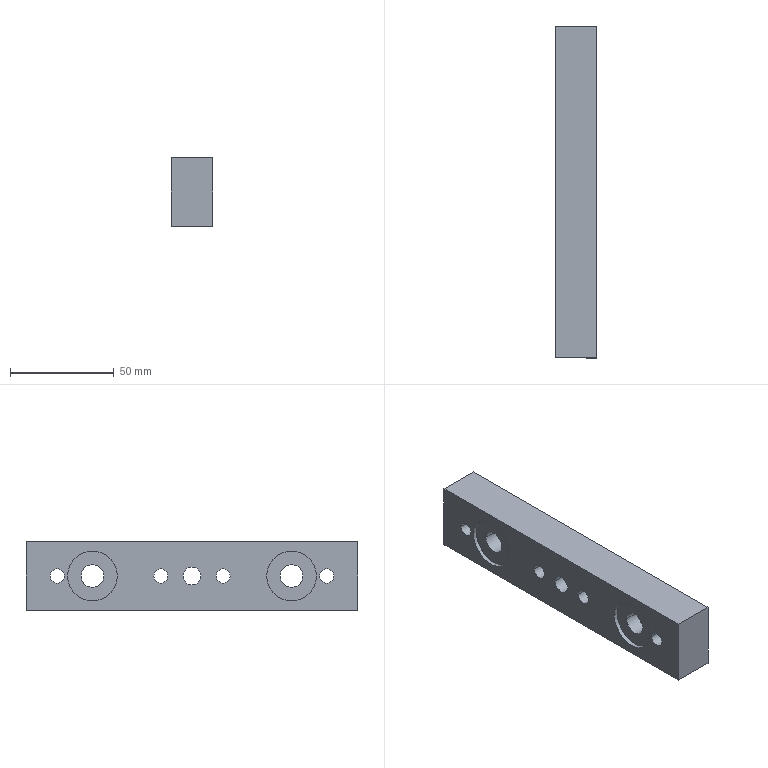Component | SolidWorks | ClampingAssembly-2_CylinderLockingBlock2-1 | 1 solid | 32 faces | box 20 x 160 x 33 mm | volume 92949 mm3 | cylinder 22 | plane 10 | commonest cylinder face diameters 6.8 x8 24 x4 18 x4 11 x4 8.5 x2 | material Q235
build123d program:
from build123d import *

# Parameters (mm, degrees)
SKETCH1_W                                        = 160
SKETCH1_H                                        = 33
BOSS_EXTRUDE1_DEPTH                              = 20
M10_TAPPED_HOLE1_D                               = 8.5
M10_TAPPED_HOLE1_DEPTH                           = 24.5
M10_TAPPED_HOLE1_TIP                             = 2.554
M10_HEX_SOCKET_HEAD_CAP_SCREW_CBORE1_D           = 11
M10_HEX_SOCKET_HEAD_CAP_SCREW_CBORE1_CBORE_D     = 18
M10_HEX_SOCKET_HEAD_CAP_SCREW_CBORE1_CBORE_DEPTH = 10.6
SKETCH7_R                                        = 12
CUT_EXTRUDE1_DEPTH                               = 2
M8_TAPPED_HOLE1_D                                = 6.8


with BuildPart() as part:
    # Sketch1 → Boss-Extrude1 (new body)
    with BuildSketch(Plane.XY):
        Rectangle(SKETCH1_W, SKETCH1_H)
    extrude(amount=BOSS_EXTRUDE1_DEPTH)

    # M10 Tapped Hole1
    with Locations(Plane.XY.offset(20)):
        with Locations((0, 0)):
            Hole(M10_TAPPED_HOLE1_D / 2, depth=M10_TAPPED_HOLE1_DEPTH)
            with Locations((0, 0, -(M10_TAPPED_HOLE1_DEPTH + M10_TAPPED_HOLE1_TIP / 2))):  # 118° drill point
                Cone(0, M10_TAPPED_HOLE1_D / 2, M10_TAPPED_HOLE1_TIP, mode=Mode.SUBTRACT)

    # M10 Hex Socket Head Cap Screw CBORE1 (through all)
    with Locations(Plane(origin=(-48, 0, 0), x_dir=(-1, 0, 0), z_dir=(0, 0, -1))):
        with Locations((0, 0)):
            m10_hex_socket_head_cap_screw_cbore1 = CounterBoreHole(M10_HEX_SOCKET_HEAD_CAP_SCREW_CBORE1_D / 2, M10_HEX_SOCKET_HEAD_CAP_SCREW_CBORE1_CBORE_D / 2, M10_HEX_SOCKET_HEAD_CAP_SCREW_CBORE1_CBORE_DEPTH)

    # Mirror1: M10 Hex Socket Head Cap Screw CBORE1 across plane
    add(m10_hex_socket_head_cap_screw_cbore1.mirror(Plane(origin=(0, 0, 0), x_dir=(0, 0, 1), z_dir=(1, 0, 0))), mode=Mode.SUBTRACT)

    # Sketch7 → Cut-Extrude1 (cut)
    with BuildSketch(Plane.XY.offset(20)):
        with Locations((-48, 0)):
            Circle(SKETCH7_R)
        with Locations((48, 0)):
            Circle(SKETCH7_R)
    extrude(amount=-CUT_EXTRUDE1_DEPTH, mode=Mode.SUBTRACT)

    # M8 Tapped Hole1 (through all)
    with Locations(Plane(origin=(65, 0, 0), x_dir=(-1, 0, 0), z_dir=(0, 0, -1))):
        with Locations((0, 0), (50, 0), (80, 0), (130, 0)):
            Hole(M8_TAPPED_HOLE1_D / 2)


solid = part.part

# Placed as in the assembly
solid = solid.moved(Location((-116.365, -26.917, -1210.457), (90, -90, 0)))
STEP:
#1=COLOUR_RGB('',0.7922,0.8196,0.9333);
#2=FILL_AREA_STYLE_COLOUR('',#1);
#3=FILL_AREA_STYLE('',(#2));
#4=SURFACE_STYLE_FILL_AREA(#3);
#5=SURFACE_SIDE_STYLE('',(#4));
#6=SURFACE_STYLE_USAGE(.BOTH.,#5);
#7=PRESENTATION_STYLE_ASSIGNMENT((#6));
#8=CARTESIAN_POINT('',(-5.369,-3.753,-47.656));
#9=VERTEX_POINT('',#8);
#10=CARTESIAN_POINT('',(-5.369,-3.485,-47.656));
#11=VERTEX_POINT('',#10);
#12=CARTESIAN_POINT('',(-5.369,-3.619,-47.656));
#13=DIRECTION('',(1.,-0.,0.));
#14=DIRECTION('',(0.,1.,0.));
#15=AXIS2_PLACEMENT_3D('',#12,#13,#14);
#16=CIRCLE('',#15,0.1339);
#17=EDGE_CURVE('',#9,#11,#16,.T.);
#18=ORIENTED_EDGE('',*,*,#17,.F.);
#19=CARTESIAN_POINT('',(-4.581,-3.753,-47.656));
#20=VERTEX_POINT('',#19);
#21=CARTESIAN_POINT('',(-4.581,-3.753,-47.656));
#22=DIRECTION('',(1.,-0.,0.));
#23=VECTOR('',#22,39.37);
#24=LINE('',#21,#23);
#25=EDGE_CURVE('',#9,#20,#24,.T.);
#26=ORIENTED_EDGE('',*,*,#25,.T.);
#27=CARTESIAN_POINT('',(-4.581,-3.485,-47.656));
#28=VERTEX_POINT('',#27);
#29=CARTESIAN_POINT('',(-4.581,-3.619,-47.656));
#30=DIRECTION('',(1.,-0.,0.));
#31=DIRECTION('',(0.,1.,0.));
#32=AXIS2_PLACEMENT_3D('',#29,#30,#31);
#33=CIRCLE('',#32,0.1339);
#34=EDGE_CURVE('',#20,#28,#33,.T.);
#35=ORIENTED_EDGE('',*,*,#34,.T.);
#36=CARTESIAN_POINT('',(-4.581,-3.485,-47.656));
#37=DIRECTION('',(1.,-0.,0.));
#38=VECTOR('',#37,39.37);
#39=LINE('',#36,#38);
#40=EDGE_CURVE('',#11,#28,#39,.T.);
#41=ORIENTED_EDGE('',*,*,#40,.F.);
#42=EDGE_LOOP('',(#18,#26,#35,#41));
#43=FACE_OUTER_BOUND('',#42,.T.);
#44=CARTESIAN_POINT('',(-4.581,-3.619,-47.656));
#45=DIRECTION('',(1.,-0.,0.));
#46=DIRECTION('',(0.,1.,0.));
#47=AXIS2_PLACEMENT_3D('',#44,#45,#46);
#48=CYLINDRICAL_SURFACE('',#47,0.1339);
#49=ADVANCED_FACE('',(#43),#48,.F.);
#50=CARTESIAN_POINT('',(-5.369,-1.784,-47.656));
#51=VERTEX_POINT('',#50);
#52=CARTESIAN_POINT('',(-5.369,-1.516,-47.656));
#53=VERTEX_POINT('',#52);
#54=CARTESIAN_POINT('',(-5.369,-1.65,-47.656));
#55=DIRECTION('',(1.,-0.,0.));
#56=DIRECTION('',(0.,1.,0.));
#57=AXIS2_PLACEMENT_3D('',#54,#55,#56);
#58=CIRCLE('',#57,0.1339);
#59=EDGE_CURVE('',#51,#53,#58,.T.);
#60=ORIENTED_EDGE('',*,*,#59,.F.);
#61=CARTESIAN_POINT('',(-4.581,-1.784,-47.656));
#62=VERTEX_POINT('',#61);
#63=CARTESIAN_POINT('',(-4.581,-1.784,-47.656));
#64=DIRECTION('',(1.,-0.,0.));
#65=VECTOR('',#64,39.37);
#66=LINE('',#63,#65);
#67=EDGE_CURVE('',#51,#62,#66,.T.);
#68=ORIENTED_EDGE('',*,*,#67,.T.);
#69=CARTESIAN_POINT('',(-4.581,-1.516,-47.656));
#70=VERTEX_POINT('',#69);
#71=CARTESIAN_POINT('',(-4.581,-1.65,-47.656));
#72=DIRECTION('',(1.,-0.,0.));
#73=DIRECTION('',(0.,1.,0.));
#74=AXIS2_PLACEMENT_3D('',#71,#72,#73);
#75=CIRCLE('',#74,0.1339);
#76=EDGE_CURVE('',#62,#70,#75,.T.);
#77=ORIENTED_EDGE('',*,*,#76,.T.);
#78=CARTESIAN_POINT('',(-4.581,-1.516,-47.656));
#79=DIRECTION('',(1.,-0.,0.));
#80=VECTOR('',#79,39.37);
#81=LINE('',#78,#80);
#82=EDGE_CURVE('',#53,#70,#81,.T.);
#83=ORIENTED_EDGE('',*,*,#82,.F.);
#84=EDGE_LOOP('',(#60,#68,#77,#83));
#85=FACE_OUTER_BOUND('',#84,.T.);
#86=CARTESIAN_POINT('',(-4.581,-1.65,-47.656));
#87=DIRECTION('',(1.,-0.,0.));
#88=DIRECTION('',(0.,1.,0.));
#89=AXIS2_PLACEMENT_3D('',#86,#87,#88);
#90=CYLINDRICAL_SURFACE('',#89,0.1339);
#91=ADVANCED_FACE('',(#85),#90,.F.);
#92=CARTESIAN_POINT('',(-5.369,-0.603,-47.656));
#93=VERTEX_POINT('',#92);
#94=CARTESIAN_POINT('',(-5.369,-0.3353,-47.656));
#95=VERTEX_POINT('',#94);
#96=CARTESIAN_POINT('',(-5.369,-0.4692,-47.656));
#97=DIRECTION('',(1.,-0.,0.));
#98=DIRECTION('',(0.,1.,0.));
#99=AXIS2_PLACEMENT_3D('',#96,#97,#98);
#100=CIRCLE('',#99,0.1339);
#101=EDGE_CURVE('',#93,#95,#100,.T.);
#102=ORIENTED_EDGE('',*,*,#101,.F.);
#103=CARTESIAN_POINT('',(-4.581,-0.603,-47.656));
#104=VERTEX_POINT('',#103);
#105=CARTESIAN_POINT('',(-4.581,-0.603,-47.656));
#106=DIRECTION('',(1.,-0.,0.));
#107=VECTOR('',#106,39.37);
#108=LINE('',#105,#107);
#109=EDGE_CURVE('',#93,#104,#108,.T.);
#110=ORIENTED_EDGE('',*,*,#109,.T.);
#111=CARTESIAN_POINT('',(-4.581,-0.3353,-47.656));
#112=VERTEX_POINT('',#111);
#113=CARTESIAN_POINT('',(-4.581,-0.4692,-47.656));
#114=DIRECTION('',(1.,-0.,0.));
#115=DIRECTION('',(0.,1.,0.));
#116=AXIS2_PLACEMENT_3D('',#113,#114,#115);
#117=CIRCLE('',#116,0.1339);
#118=EDGE_CURVE('',#104,#112,#117,.T.);
#119=ORIENTED_EDGE('',*,*,#118,.T.);
#120=CARTESIAN_POINT('',(-4.581,-0.3353,-47.656));
#121=DIRECTION('',(1.,-0.,0.));
#122=VECTOR('',#121,39.37);
#123=LINE('',#120,#122);
#124=EDGE_CURVE('',#95,#112,#123,.T.);
#125=ORIENTED_EDGE('',*,*,#124,.F.);
#126=EDGE_LOOP('',(#102,#110,#119,#125));
#127=FACE_OUTER_BOUND('',#126,.T.);
#128=CARTESIAN_POINT('',(-4.581,-0.4692,-47.656));
#129=DIRECTION('',(1.,-0.,0.));
#130=DIRECTION('',(0.,1.,0.));
#131=AXIS2_PLACEMENT_3D('',#128,#129,#130);
#132=CYLINDRICAL_SURFACE('',#131,0.1339);
#133=ADVANCED_FACE('',(#127),#132,.F.);
#134=CARTESIAN_POINT('',(-5.369,1.365,-47.656));
#135=VERTEX_POINT('',#134);
#136=CARTESIAN_POINT('',(-5.369,1.633,-47.656));
#137=VERTEX_POINT('',#136);
#138=CARTESIAN_POINT('',(-5.369,1.499,-47.656));
#139=DIRECTION('',(1.,-0.,0.));
#140=DIRECTION('',(0.,1.,0.));
#141=AXIS2_PLACEMENT_3D('',#138,#139,#140);
#142=CIRCLE('',#141,0.1339);
#143=EDGE_CURVE('',#135,#137,#142,.T.);
#144=ORIENTED_EDGE('',*,*,#143,.F.);
#145=CARTESIAN_POINT('',(-4.581,1.365,-47.656));
#146=VERTEX_POINT('',#145);
#147=CARTESIAN_POINT('',(-4.581,1.365,-47.656));
#148=DIRECTION('',(1.,-0.,0.));
#149=VECTOR('',#148,39.37);
#150=LINE('',#147,#149);
#151=EDGE_CURVE('',#135,#146,#150,.T.);
#152=ORIENTED_EDGE('',*,*,#151,.T.);
#153=CARTESIAN_POINT('',(-4.581,1.633,-47.656));
#154=VERTEX_POINT('',#153);
#155=CARTESIAN_POINT('',(-4.581,1.499,-47.656));
#156=DIRECTION('',(1.,-0.,0.));
#157=DIRECTION('',(0.,1.,0.));
#158=AXIS2_PLACEMENT_3D('',#155,#156,#157);
#159=CIRCLE('',#158,0.1339);
#160=EDGE_CURVE('',#146,#154,#159,.T.);
#161=ORIENTED_EDGE('',*,*,#160,.T.);
#162=CARTESIAN_POINT('',(-4.581,1.633,-47.656));
#163=DIRECTION('',(1.,-0.,0.));
#164=VECTOR('',#163,39.37);
#165=LINE('',#162,#164);
#166=EDGE_CURVE('',#137,#154,#165,.T.);
#167=ORIENTED_EDGE('',*,*,#166,.F.);
#168=EDGE_LOOP('',(#144,#152,#161,#167));
#169=FACE_OUTER_BOUND('',#168,.T.);
#170=CARTESIAN_POINT('',(-4.581,1.499,-47.656));
#171=DIRECTION('',(1.,-0.,0.));
#172=DIRECTION('',(0.,1.,0.));
#173=AXIS2_PLACEMENT_3D('',#170,#171,#172);
#174=CYLINDRICAL_SURFACE('',#173,0.1339);
#175=ADVANCED_FACE('',(#169),#174,.F.);
#176=CARTESIAN_POINT('',(-5.29,-2.477,-47.656));
#177=VERTEX_POINT('',#176);
#178=CARTESIAN_POINT('',(-5.29,-3.422,-47.656));
#179=VERTEX_POINT('',#178);
#180=CARTESIAN_POINT('',(-5.29,-2.949,-47.656));
#181=DIRECTION('',(-1.,0.,-0.));
#182=DIRECTION('',(0.,-1.,0.));
#183=AXIS2_PLACEMENT_3D('',#180,#181,#182);
#184=CIRCLE('',#183,0.4724);
#185=EDGE_CURVE('',#177,#179,#184,.T.);
#186=ORIENTED_EDGE('',*,*,#185,.F.);
#187=CARTESIAN_POINT('',(-5.369,-2.477,-47.656));
#188=VERTEX_POINT('',#187);
#189=CARTESIAN_POINT('',(-5.29,-2.477,-47.656));
#190=DIRECTION('',(-1.,0.,-0.));
#191=VECTOR('',#190,39.37);
#192=LINE('',#189,#191);
#193=EDGE_CURVE('',#177,#188,#192,.T.);
#194=ORIENTED_EDGE('',*,*,#193,.T.);
#195=CARTESIAN_POINT('',(-5.369,-3.422,-47.656));
#196=VERTEX_POINT('',#195);
#197=CARTESIAN_POINT('',(-5.369,-2.949,-47.656));
#198=DIRECTION('',(-1.,0.,-0.));
#199=DIRECTION('',(0.,-1.,0.));
#200=AXIS2_PLACEMENT_3D('',#197,#198,#199);
#201=CIRCLE('',#200,0.4724);
#202=EDGE_CURVE('',#188,#196,#201,.T.);
#203=ORIENTED_EDGE('',*,*,#202,.T.);
#204=CARTESIAN_POINT('',(-5.29,-3.422,-47.656));
#205=DIRECTION('',(-1.,0.,-0.));
#206=VECTOR('',#205,39.37);
#207=LINE('',#204,#206);
#208=EDGE_CURVE('',#179,#196,#207,.T.);
#209=ORIENTED_EDGE('',*,*,#208,.F.);
#210=EDGE_LOOP('',(#186,#194,#203,#209));
#211=FACE_OUTER_BOUND('',#210,.T.);
#212=CARTESIAN_POINT('',(-5.29,-2.949,-47.656));
#213=DIRECTION('',(-1.,0.,-0.));
#214=DIRECTION('',(0.,-1.,0.));
#215=AXIS2_PLACEMENT_3D('',#212,#213,#214);
#216=CYLINDRICAL_SURFACE('',#215,0.4724);
#217=ADVANCED_FACE('',(#211),#216,.F.);
#218=CARTESIAN_POINT('',(-5.29,1.302,-47.656));
#219=VERTEX_POINT('',#218);
#220=CARTESIAN_POINT('',(-5.29,0.3576,-47.656));
#221=VERTEX_POINT('',#220);
#222=CARTESIAN_POINT('',(-5.29,0.83,-47.656));
#223=DIRECTION('',(-1.,0.,-0.));
#224=DIRECTION('',(0.,-1.,0.));
#225=AXIS2_PLACEMENT_3D('',#222,#223,#224);
#226=CIRCLE('',#225,0.4724);
#227=EDGE_CURVE('',#219,#221,#226,.T.);
#228=ORIENTED_EDGE('',*,*,#227,.F.);
#229=CARTESIAN_POINT('',(-5.369,1.302,-47.656));
#230=VERTEX_POINT('',#229);
#231=CARTESIAN_POINT('',(-5.29,1.302,-47.656));
#232=DIRECTION('',(-1.,0.,-0.));
#233=VECTOR('',#232,39.37);
#234=LINE('',#231,#233);
#235=EDGE_CURVE('',#219,#230,#234,.T.);
#236=ORIENTED_EDGE('',*,*,#235,.T.);
#237=CARTESIAN_POINT('',(-5.369,0.3576,-47.656));
#238=VERTEX_POINT('',#237);
#239=CARTESIAN_POINT('',(-5.369,0.83,-47.656));
#240=DIRECTION('',(-1.,0.,-0.));
#241=DIRECTION('',(0.,-1.,0.));
#242=AXIS2_PLACEMENT_3D('',#239,#240,#241);
#243=CIRCLE('',#242,0.4724);
#244=EDGE_CURVE('',#230,#238,#243,.T.);
#245=ORIENTED_EDGE('',*,*,#244,.T.);
#246=CARTESIAN_POINT('',(-5.29,0.3576,-47.656));
#247=DIRECTION('',(-1.,0.,-0.));
#248=VECTOR('',#247,39.37);
#249=LINE('',#246,#248);
#250=EDGE_CURVE('',#221,#238,#249,.T.);
#251=ORIENTED_EDGE('',*,*,#250,.F.);
#252=EDGE_LOOP('',(#228,#236,#245,#251));
#253=FACE_OUTER_BOUND('',#252,.T.);
#254=CARTESIAN_POINT('',(-5.29,0.83,-47.656));
#255=DIRECTION('',(-1.,0.,-0.));
#256=DIRECTION('',(0.,-1.,0.));
#257=AXIS2_PLACEMENT_3D('',#254,#255,#256);
#258=CYLINDRICAL_SURFACE('',#257,0.4724);
#259=ADVANCED_FACE('',(#253),#258,.F.);
#260=CARTESIAN_POINT('',(-4.999,-3.304,-47.656));
#261=VERTEX_POINT('',#260);
#262=CARTESIAN_POINT('',(-4.999,-2.595,-47.656));
#263=VERTEX_POINT('',#262);
#264=CARTESIAN_POINT('',(-4.999,-2.949,-47.656));
#265=DIRECTION('',(1.,-0.,0.));
#266=DIRECTION('',(0.,1.,0.));
#267=AXIS2_PLACEMENT_3D('',#264,#265,#266);
#268=CIRCLE('',#267,0.3543);
#269=EDGE_CURVE('',#261,#263,#268,.T.);
#270=ORIENTED_EDGE('',*,*,#269,.F.);
#271=CARTESIAN_POINT('',(-4.581,-3.304,-47.656));
#272=VERTEX_POINT('',#271);
#273=CARTESIAN_POINT('',(-4.581,-3.304,-47.656));
#274=DIRECTION('',(1.,-0.,0.));
#275=VECTOR('',#274,39.37);
#276=LINE('',#273,#275);
#277=EDGE_CURVE('',#261,#272,#276,.T.);
#278=ORIENTED_EDGE('',*,*,#277,.T.);
#279=CARTESIAN_POINT('',(-4.581,-2.595,-47.656));
#280=VERTEX_POINT('',#279);
#281=CARTESIAN_POINT('',(-4.581,-2.949,-47.656));
#282=DIRECTION('',(1.,-0.,0.));
#283=DIRECTION('',(0.,1.,0.));
#284=AXIS2_PLACEMENT_3D('',#281,#282,#283);
#285=CIRCLE('',#284,0.3543);
#286=EDGE_CURVE('',#272,#280,#285,.T.);
#287=ORIENTED_EDGE('',*,*,#286,.T.);
#288=CARTESIAN_POINT('',(-4.581,-2.595,-47.656));
#289=DIRECTION('',(1.,-0.,0.));
#290=VECTOR('',#289,39.37);
#291=LINE('',#288,#290);
#292=EDGE_CURVE('',#263,#280,#291,.T.);
#293=ORIENTED_EDGE('',*,*,#292,.F.);
#294=EDGE_LOOP('',(#270,#278,#287,#293));
#295=FACE_OUTER_BOUND('',#294,.T.);
#296=CARTESIAN_POINT('',(-4.581,-2.949,-47.656));
#297=DIRECTION('',(1.,-0.,0.));
#298=DIRECTION('',(0.,1.,0.));
#299=AXIS2_PLACEMENT_3D('',#296,#297,#298);
#300=CYLINDRICAL_SURFACE('',#299,0.3543);
#301=ADVANCED_FACE('',(#295),#300,.F.);
#302=CARTESIAN_POINT('',(-4.999,0.4757,-47.656));
#303=VERTEX_POINT('',#302);
#304=CARTESIAN_POINT('',(-4.999,1.184,-47.656));
#305=VERTEX_POINT('',#304);
#306=CARTESIAN_POINT('',(-4.999,0.83,-47.656));
#307=DIRECTION('',(1.,-0.,0.));
#308=DIRECTION('',(0.,1.,0.));
#309=AXIS2_PLACEMENT_3D('',#306,#307,#308);
#310=CIRCLE('',#309,0.3543);
#311=EDGE_CURVE('',#303,#305,#310,.T.);
#312=ORIENTED_EDGE('',*,*,#311,.F.);
#313=CARTESIAN_POINT('',(-4.581,0.4757,-47.656));
#314=VERTEX_POINT('',#313);
#315=CARTESIAN_POINT('',(-4.581,0.4757,-47.656));
#316=DIRECTION('',(1.,-0.,0.));
#317=VECTOR('',#316,39.37);
#318=LINE('',#315,#317);
#319=EDGE_CURVE('',#303,#314,#318,.T.);
#320=ORIENTED_EDGE('',*,*,#319,.T.);
#321=CARTESIAN_POINT('',(-4.581,1.184,-47.656));
#322=VERTEX_POINT('',#321);
#323=CARTESIAN_POINT('',(-4.581,0.83,-47.656));
#324=DIRECTION('',(1.,-0.,0.));
#325=DIRECTION('',(0.,1.,0.));
#326=AXIS2_PLACEMENT_3D('',#323,#324,#325);
#327=CIRCLE('',#326,0.3543);
#328=EDGE_CURVE('',#314,#322,#327,.T.);
#329=ORIENTED_EDGE('',*,*,#328,.T.);
#330=CARTESIAN_POINT('',(-4.581,1.184,-47.656));
#331=DIRECTION('',(1.,-0.,0.));
#332=VECTOR('',#331,39.37);
#333=LINE('',#330,#332);
#334=EDGE_CURVE('',#305,#322,#333,.T.);
#335=ORIENTED_EDGE('',*,*,#334,.F.);
#336=EDGE_LOOP('',(#312,#320,#329,#335));
#337=FACE_OUTER_BOUND('',#336,.T.);
#338=CARTESIAN_POINT('',(-4.581,0.83,-47.656));
#339=DIRECTION('',(1.,-0.,0.));
#340=DIRECTION('',(0.,1.,0.));
#341=AXIS2_PLACEMENT_3D('',#338,#339,#340);
#342=CYLINDRICAL_SURFACE('',#341,0.3543);
#343=ADVANCED_FACE('',(#337),#342,.F.);
#344=CARTESIAN_POINT('',(-4.581,-0.8924,-47.656));
#345=VERTEX_POINT('',#344);
#346=CARTESIAN_POINT('',(-4.581,-1.227,-47.656));
#347=VERTEX_POINT('',#346);
#348=CARTESIAN_POINT('',(-4.581,-1.06,-47.656));
#349=DIRECTION('',(-1.,0.,-0.));
#350=DIRECTION('',(0.,-1.,0.));
#351=AXIS2_PLACEMENT_3D('',#348,#349,#350);
#352=CIRCLE('',#351,0.1673);
#353=EDGE_CURVE('',#345,#347,#352,.T.);
#354=ORIENTED_EDGE('',*,*,#353,.F.);
#355=CARTESIAN_POINT('',(-5.369,-0.8924,-47.656));
#356=VERTEX_POINT('',#355);
#357=CARTESIAN_POINT('',(-5.369,-0.8924,-47.656));
#358=DIRECTION('',(-1.,0.,-0.));
#359=VECTOR('',#358,39.37);
#360=LINE('',#357,#359);
#361=EDGE_CURVE('',#345,#356,#360,.T.);
#362=ORIENTED_EDGE('',*,*,#361,.T.);
#363=CARTESIAN_POINT('',(-5.369,-1.227,-47.656));
#364=VERTEX_POINT('',#363);
#365=CARTESIAN_POINT('',(-5.369,-1.06,-47.656));
#366=DIRECTION('',(-1.,0.,-0.));
#367=DIRECTION('',(0.,-1.,0.));
#368=AXIS2_PLACEMENT_3D('',#365,#366,#367);
#369=CIRCLE('',#368,0.1673);
#370=EDGE_CURVE('',#356,#364,#369,.T.);
#371=ORIENTED_EDGE('',*,*,#370,.T.);
#372=CARTESIAN_POINT('',(-5.369,-1.227,-47.656));
#373=DIRECTION('',(-1.,0.,-0.));
#374=VECTOR('',#373,39.37);
#375=LINE('',#372,#374);
#376=EDGE_CURVE('',#347,#364,#375,.T.);
#377=ORIENTED_EDGE('',*,*,#376,.F.);
#378=EDGE_LOOP('',(#354,#362,#371,#377));
#379=FACE_OUTER_BOUND('',#378,.T.);
#380=CARTESIAN_POINT('',(-5.369,-1.06,-47.656));
#381=DIRECTION('',(-1.,0.,-0.));
#382=DIRECTION('',(0.,-1.,0.));
#383=AXIS2_PLACEMENT_3D('',#380,#381,#382);
#384=CYLINDRICAL_SURFACE('',#383,0.1673);
#385=ADVANCED_FACE('',(#379),#384,.F.);
#386=CARTESIAN_POINT('',(-5.29,0.6135,-47.656));
#387=VERTEX_POINT('',#386);
#388=CARTESIAN_POINT('',(-5.29,1.047,-47.656));
#389=VERTEX_POINT('',#388);
#390=CARTESIAN_POINT('',(-5.29,0.83,-47.656));
#391=DIRECTION('',(1.,-0.,0.));
#392=DIRECTION('',(0.,-1.,0.));
#393=AXIS2_PLACEMENT_3D('',#390,#391,#392);
#394=CIRCLE('',#393,0.2165);
#395=EDGE_CURVE('',#387,#389,#394,.T.);
#396=ORIENTED_EDGE('',*,*,#395,.F.);
#397=CARTESIAN_POINT('',(-4.999,0.6135,-47.656));
#398=VERTEX_POINT('',#397);
#399=CARTESIAN_POINT('',(-4.581,0.6135,-47.656));
#400=DIRECTION('',(1.,-0.,0.));
#401=VECTOR('',#400,39.37);
#402=LINE('',#399,#401);
#403=EDGE_CURVE('',#387,#398,#402,.T.);
#404=ORIENTED_EDGE('',*,*,#403,.T.);
#405=CARTESIAN_POINT('',(-4.999,1.047,-47.656));
#406=VERTEX_POINT('',#405);
#407=CARTESIAN_POINT('',(-4.999,0.83,-47.656));
#408=DIRECTION('',(1.,-0.,0.));
#409=DIRECTION('',(0.,1.,0.));
#410=AXIS2_PLACEMENT_3D('',#407,#408,#409);
#411=CIRCLE('',#410,0.2165);
#412=EDGE_CURVE('',#398,#406,#411,.T.);
#413=ORIENTED_EDGE('',*,*,#412,.T.);
#414=CARTESIAN_POINT('',(-4.581,1.047,-47.656));
#415=DIRECTION('',(1.,-0.,0.));
#416=VECTOR('',#415,39.37);
#417=LINE('',#414,#416);
#418=EDGE_CURVE('',#389,#406,#417,.T.);
#419=ORIENTED_EDGE('',*,*,#418,.F.);
#420=EDGE_LOOP('',(#396,#404,#413,#419));
#421=FACE_OUTER_BOUND('',#420,.T.);
#422=CARTESIAN_POINT('',(-4.581,0.83,-47.656));
#423=DIRECTION('',(1.,-0.,0.));
#424=DIRECTION('',(0.,1.,0.));
#425=AXIS2_PLACEMENT_3D('',#422,#423,#424);
#426=CYLINDRICAL_SURFACE('',#425,0.2165);
#427=ADVANCED_FACE('',(#421),#426,.F.);
#428=CARTESIAN_POINT('',(-5.29,-3.166,-47.656));
#429=VERTEX_POINT('',#428);
#430=CARTESIAN_POINT('',(-5.29,-2.733,-47.656));
#431=VERTEX_POINT('',#430);
#432=CARTESIAN_POINT('',(-5.29,-2.949,-47.656));
#433=DIRECTION('',(1.,-0.,0.));
#434=DIRECTION('',(0.,-1.,0.));
#435=AXIS2_PLACEMENT_3D('',#432,#433,#434);
#436=CIRCLE('',#435,0.2165);
#437=EDGE_CURVE('',#429,#431,#436,.T.);
#438=ORIENTED_EDGE('',*,*,#437,.F.);
#439=CARTESIAN_POINT('',(-4.999,-3.166,-47.656));
#440=VERTEX_POINT('',#439);
#441=CARTESIAN_POINT('',(-4.581,-3.166,-47.656));
#442=DIRECTION('',(1.,-0.,0.));
#443=VECTOR('',#442,39.37);
#444=LINE('',#441,#443);
#445=EDGE_CURVE('',#429,#440,#444,.T.);
#446=ORIENTED_EDGE('',*,*,#445,.T.);
#447=CARTESIAN_POINT('',(-4.999,-2.733,-47.656));
#448=VERTEX_POINT('',#447);
#449=CARTESIAN_POINT('',(-4.999,-2.949,-47.656));
#450=DIRECTION('',(1.,-0.,0.));
#451=DIRECTION('',(0.,1.,0.));
#452=AXIS2_PLACEMENT_3D('',#449,#450,#451);
#453=CIRCLE('',#452,0.2165);
#454=EDGE_CURVE('',#440,#448,#453,.T.);
#455=ORIENTED_EDGE('',*,*,#454,.T.);
#456=CARTESIAN_POINT('',(-4.581,-2.733,-47.656));
#457=DIRECTION('',(1.,-0.,0.));
#458=VECTOR('',#457,39.37);
#459=LINE('',#456,#458);
#460=EDGE_CURVE('',#431,#448,#459,.T.);
#461=ORIENTED_EDGE('',*,*,#460,.F.);
#462=EDGE_LOOP('',(#438,#446,#455,#461));
#463=FACE_OUTER_BOUND('',#462,.T.);
#464=CARTESIAN_POINT('',(-4.581,-2.949,-47.656));
#465=DIRECTION('',(1.,-0.,0.));
#466=DIRECTION('',(0.,1.,0.));
#467=AXIS2_PLACEMENT_3D('',#464,#465,#466);
#468=CYLINDRICAL_SURFACE('',#467,0.2165);
#469=ADVANCED_FACE('',(#463),#468,.F.);
#470=ORIENTED_EDGE('',*,*,#445,.F.);
#471=CARTESIAN_POINT('',(-5.29,-2.949,-47.656));
#472=DIRECTION('',(1.,-0.,0.));
#473=DIRECTION('',(0.,-1.,0.));
#474=AXIS2_PLACEMENT_3D('',#471,#472,#473);
#475=CIRCLE('',#474,0.2165);
#476=EDGE_CURVE('',#431,#429,#475,.T.);
#477=ORIENTED_EDGE('',*,*,#476,.F.);
#478=ORIENTED_EDGE('',*,*,#460,.T.);
#479=CARTESIAN_POINT('',(-4.999,-2.949,-47.656));
#480=DIRECTION('',(1.,-0.,0.));
#481=DIRECTION('',(0.,1.,0.));
#482=AXIS2_PLACEMENT_3D('',#479,#480,#481);
#483=CIRCLE('',#482,0.2165);
#484=EDGE_CURVE('',#448,#440,#483,.T.);
#485=ORIENTED_EDGE('',*,*,#484,.T.);
#486=EDGE_LOOP('',(#470,#477,#478,#485));
#487=FACE_OUTER_BOUND('',#486,.T.);
#488=CARTESIAN_POINT('',(-4.581,-2.949,-47.656));
#489=DIRECTION('',(1.,-0.,0.));
#490=DIRECTION('',(0.,1.,0.));
#491=AXIS2_PLACEMENT_3D('',#488,#489,#490);
#492=CYLINDRICAL_SURFACE('',#491,0.2165);
#493=ADVANCED_FACE('',(#487),#492,.F.);
#494=ORIENTED_EDGE('',*,*,#403,.F.);
#495=CARTESIAN_POINT('',(-5.29,0.83,-47.656));
#496=DIRECTION('',(1.,-0.,0.));
#497=DIRECTION('',(0.,-1.,0.));
#498=AXIS2_PLACEMENT_3D('',#495,#496,#497);
#499=CIRCLE('',#498,0.2165);
#500=EDGE_CURVE('',#389,#387,#499,.T.);
#501=ORIENTED_EDGE('',*,*,#500,.F.);
#502=ORIENTED_EDGE('',*,*,#418,.T.);
#503=CARTESIAN_POINT('',(-4.999,0.83,-47.656));
#504=DIRECTION('',(1.,-0.,0.));
#505=DIRECTION('',(0.,1.,0.));
#506=AXIS2_PLACEMENT_3D('',#503,#504,#505);
#507=CIRCLE('',#506,0.2165);
#508=EDGE_CURVE('',#406,#398,#507,.T.);
#509=ORIENTED_EDGE('',*,*,#508,.T.);
#510=EDGE_LOOP('',(#494,#501,#502,#509));
#511=FACE_OUTER_BOUND('',#510,.T.);
#512=CARTESIAN_POINT('',(-4.581,0.83,-47.656));
#513=DIRECTION('',(1.,-0.,0.));
#514=DIRECTION('',(0.,1.,0.));
#515=AXIS2_PLACEMENT_3D('',#512,#513,#514);
#516=CYLINDRICAL_SURFACE('',#515,0.2165);
#517=ADVANCED_FACE('',(#511),#516,.F.);
#518=CARTESIAN_POINT('',(-4.581,-4.209,-48.305));
#519=VERTEX_POINT('',#518);
#520=CARTESIAN_POINT('',(-4.581,-4.209,-47.006));
#521=VERTEX_POINT('',#520);
#522=CARTESIAN_POINT('',(-4.581,-4.209,-47.006));
#523=DIRECTION('',(-0.,-0.,1.));
#524=VECTOR('',#523,39.37);
#525=LINE('',#522,#524);
#526=EDGE_CURVE('',#519,#521,#525,.T.);
#527=ORIENTED_EDGE('',*,*,#526,.T.);
#528=CARTESIAN_POINT('',(-5.369,-4.209,-47.006));
#529=VERTEX_POINT('',#528);
#530=CARTESIAN_POINT('',(-5.369,-4.209,-47.006));
#531=DIRECTION('',(1.,-0.,0.));
#532=VECTOR('',#531,39.37);
#533=LINE('',#530,#532);
#534=EDGE_CURVE('',#529,#521,#533,.T.);
#535=ORIENTED_EDGE('',*,*,#534,.F.);
#536=CARTESIAN_POINT('',(-5.369,-4.209,-48.305));
#537=VERTEX_POINT('',#536);
#538=CARTESIAN_POINT('',(-5.369,-4.209,-47.006));
#539=DIRECTION('',(-0.,-0.,1.));
#540=VECTOR('',#539,39.37);
#541=LINE('',#538,#540);
#542=EDGE_CURVE('',#537,#529,#541,.T.);
#543=ORIENTED_EDGE('',*,*,#542,.F.);
#544=CARTESIAN_POINT('',(-5.369,-4.209,-48.305));
#545=DIRECTION('',(1.,-0.,0.));
#546=VECTOR('',#545,39.37);
#547=LINE('',#544,#546);
#548=EDGE_CURVE('',#537,#519,#547,.T.);
#549=ORIENTED_EDGE('',*,*,#548,.T.);
#550=EDGE_LOOP('',(#527,#535,#543,#549));
#551=FACE_OUTER_BOUND('',#550,.T.);
#552=CARTESIAN_POINT('',(-5.369,-4.209,-47.006));
#553=DIRECTION('',(0.,1.,0.));
#554=DIRECTION('',(-1.,0.,-0.));
#555=AXIS2_PLACEMENT_3D('',#552,#553,#554);
#556=PLANE('',#555);
#557=ADVANCED_FACE('',(#551),#556,.F.);
#558=CARTESIAN_POINT('',(-4.581,2.09,-47.006));
#559=VERTEX_POINT('',#558);
#560=CARTESIAN_POINT('',(-4.581,2.09,-47.006));
#561=DIRECTION('',(0.,1.,0.));
#562=VECTOR('',#561,39.37);
#563=LINE('',#560,#562);
#564=EDGE_CURVE('',#521,#559,#563,.T.);
#565=ORIENTED_EDGE('',*,*,#564,.T.);
#566=CARTESIAN_POINT('',(-5.369,2.09,-47.006));
#567=VERTEX_POINT('',#566);
#568=CARTESIAN_POINT('',(-5.369,2.09,-47.006));
#569=DIRECTION('',(1.,-0.,0.));
#570=VECTOR('',#569,39.37);
#571=LINE('',#568,#570);
#572=EDGE_CURVE('',#567,#559,#571,.T.);
#573=ORIENTED_EDGE('',*,*,#572,.F.);
#574=CARTESIAN_POINT('',(-5.369,2.09,-47.006));
#575=DIRECTION('',(0.,1.,0.));
#576=VECTOR('',#575,39.37);
#577=LINE('',#574,#576);
#578=EDGE_CURVE('',#529,#567,#577,.T.);
#579=ORIENTED_EDGE('',*,*,#578,.F.);
#580=ORIENTED_EDGE('',*,*,#534,.T.);
#581=EDGE_LOOP('',(#565,#573,#579,#580));
#582=FACE_OUTER_BOUND('',#581,.T.);
#583=CARTESIAN_POINT('',(-5.369,2.09,-47.006));
#584=DIRECTION('',(0.,0.,-1.));
#585=DIRECTION('',(1.,-0.,0.));
#586=AXIS2_PLACEMENT_3D('',#583,#584,#585);
#587=PLANE('',#586);
#588=ADVANCED_FACE('',(#582),#587,.F.);
#589=CARTESIAN_POINT('',(-4.581,2.09,-48.305));
#590=VERTEX_POINT('',#589);
#591=CARTESIAN_POINT('',(-4.581,2.09,-47.006));
#592=DIRECTION('',(0.,0.,-1.));
#593=VECTOR('',#592,39.37);
#594=LINE('',#591,#593);
#595=EDGE_CURVE('',#559,#590,#594,.T.);
#596=ORIENTED_EDGE('',*,*,#595,.T.);
#597=CARTESIAN_POINT('',(-5.369,2.09,-48.305));
#598=VERTEX_POINT('',#597);
#599=CARTESIAN_POINT('',(-5.369,2.09,-48.305));
#600=DIRECTION('',(1.,-0.,0.));
#601=VECTOR('',#600,39.37);
#602=LINE('',#599,#601);
#603=EDGE_CURVE('',#598,#590,#602,.T.);
#604=ORIENTED_EDGE('',*,*,#603,.F.);
#605=CARTESIAN_POINT('',(-5.369,2.09,-47.006));
#606=DIRECTION('',(0.,0.,-1.));
#607=VECTOR('',#606,39.37);
#608=LINE('',#605,#607);
#609=EDGE_CURVE('',#567,#598,#608,.T.);
#610=ORIENTED_EDGE('',*,*,#609,.F.);
#611=ORIENTED_EDGE('',*,*,#572,.T.);
#612=EDGE_LOOP('',(#596,#604,#610,#611));
#613=FACE_OUTER_BOUND('',#612,.T.);
#614=CARTESIAN_POINT('',(-5.369,2.09,-47.006));
#615=DIRECTION('',(-0.,-1.,-0.));
#616=DIRECTION('',(1.,-0.,0.));
#617=AXIS2_PLACEMENT_3D('',#614,#615,#616);
#618=PLANE('',#617);
#619=ADVANCED_FACE('',(#613),#618,.F.);
#620=CARTESIAN_POINT('',(-4.581,2.09,-48.305));
#621=DIRECTION('',(-0.,-1.,-0.));
#622=VECTOR('',#621,39.37);
#623=LINE('',#620,#622);
#624=EDGE_CURVE('',#590,#519,#623,.T.);
#625=ORIENTED_EDGE('',*,*,#624,.T.);
#626=ORIENTED_EDGE('',*,*,#548,.F.);
#627=CARTESIAN_POINT('',(-5.369,2.09,-48.305));
#628=DIRECTION('',(-0.,-1.,-0.));
#629=VECTOR('',#628,39.37);
#630=LINE('',#627,#629);
#631=EDGE_CURVE('',#598,#537,#630,.T.);
#632=ORIENTED_EDGE('',*,*,#631,.F.);
#633=ORIENTED_EDGE('',*,*,#603,.T.);
#634=EDGE_LOOP('',(#625,#626,#632,#633));
#635=FACE_OUTER_BOUND('',#634,.T.);
#636=CARTESIAN_POINT('',(-5.369,2.09,-48.305));
#637=DIRECTION('',(-0.,-0.,1.));
#638=DIRECTION('',(-1.,0.,-0.));
#639=AXIS2_PLACEMENT_3D('',#636,#637,#638);
#640=PLANE('',#639);
#641=ADVANCED_FACE('',(#635),#640,.F.);
#642=CARTESIAN_POINT('',(-5.369,-3.619,-47.656));
#643=DIRECTION('',(1.,-0.,0.));
#644=DIRECTION('',(0.,1.,0.));
#645=AXIS2_PLACEMENT_3D('',#642,#643,#644);
#646=CIRCLE('',#645,0.1339);
#647=EDGE_CURVE('',#11,#9,#646,.T.);
#648=ORIENTED_EDGE('',*,*,#647,.T.);
#649=ORIENTED_EDGE('',*,*,#17,.T.);
#650=EDGE_LOOP('',(#648,#649));
#651=FACE_BOUND('',#650,.T.);
#652=CARTESIAN_POINT('',(-5.369,-1.65,-47.656));
#653=DIRECTION('',(1.,-0.,0.));
#654=DIRECTION('',(0.,1.,0.));
#655=AXIS2_PLACEMENT_3D('',#652,#653,#654);
#656=CIRCLE('',#655,0.1339);
#657=EDGE_CURVE('',#53,#51,#656,.T.);
#658=ORIENTED_EDGE('',*,*,#657,.T.);
#659=ORIENTED_EDGE('',*,*,#59,.T.);
#660=EDGE_LOOP('',(#658,#659));
#661=FACE_BOUND('',#660,.T.);
#662=CARTESIAN_POINT('',(-5.369,-0.4692,-47.656));
#663=DIRECTION('',(1.,-0.,0.));
#664=DIRECTION('',(0.,1.,0.));
#665=AXIS2_PLACEMENT_3D('',#662,#663,#664);
#666=CIRCLE('',#665,0.1339);
#667=EDGE_CURVE('',#95,#93,#666,.T.);
#668=ORIENTED_EDGE('',*,*,#667,.T.);
#669=ORIENTED_EDGE('',*,*,#101,.T.);
#670=EDGE_LOOP('',(#668,#669));
#671=FACE_BOUND('',#670,.T.);
#672=CARTESIAN_POINT('',(-5.369,1.499,-47.656));
#673=DIRECTION('',(1.,-0.,0.));
#674=DIRECTION('',(0.,1.,0.));
#675=AXIS2_PLACEMENT_3D('',#672,#673,#674);
#676=CIRCLE('',#675,0.1339);
#677=EDGE_CURVE('',#137,#135,#676,.T.);
#678=ORIENTED_EDGE('',*,*,#677,.T.);
#679=ORIENTED_EDGE('',*,*,#143,.T.);
#680=EDGE_LOOP('',(#678,#679));
#681=FACE_BOUND('',#680,.T.);
#682=CARTESIAN_POINT('',(-5.369,-2.949,-47.656));
#683=DIRECTION('',(-1.,0.,-0.));
#684=DIRECTION('',(0.,-1.,0.));
#685=AXIS2_PLACEMENT_3D('',#682,#683,#684);
#686=CIRCLE('',#685,0.4724);
#687=EDGE_CURVE('',#196,#188,#686,.T.);
#688=ORIENTED_EDGE('',*,*,#687,.F.);
#689=ORIENTED_EDGE('',*,*,#202,.F.);
#690=EDGE_LOOP('',(#688,#689));
#691=FACE_BOUND('',#690,.T.);
#692=CARTESIAN_POINT('',(-5.369,0.83,-47.656));
#693=DIRECTION('',(-1.,0.,-0.));
#694=DIRECTION('',(0.,-1.,0.));
#695=AXIS2_PLACEMENT_3D('',#692,#693,#694);
#696=CIRCLE('',#695,0.4724);
#697=EDGE_CURVE('',#238,#230,#696,.T.);
#698=ORIENTED_EDGE('',*,*,#697,.F.);
#699=ORIENTED_EDGE('',*,*,#244,.F.);
#700=EDGE_LOOP('',(#698,#699));
#701=FACE_BOUND('',#700,.T.);
#702=CARTESIAN_POINT('',(-5.369,-1.06,-47.656));
#703=DIRECTION('',(-1.,0.,-0.));
#704=DIRECTION('',(0.,-1.,0.));
#705=AXIS2_PLACEMENT_3D('',#702,#703,#704);
#706=CIRCLE('',#705,0.1673);
#707=EDGE_CURVE('',#364,#356,#706,.T.);
#708=ORIENTED_EDGE('',*,*,#707,.F.);
#709=ORIENTED_EDGE('',*,*,#370,.F.);
#710=EDGE_LOOP('',(#708,#709));
#711=FACE_BOUND('',#710,.T.);
#712=ORIENTED_EDGE('',*,*,#542,.T.);
#713=ORIENTED_EDGE('',*,*,#578,.T.);
#714=ORIENTED_EDGE('',*,*,#609,.T.);
#715=ORIENTED_EDGE('',*,*,#631,.T.);
#716=EDGE_LOOP('',(#712,#713,#714,#715));
#717=FACE_OUTER_BOUND('',#716,.T.);
#718=CARTESIAN_POINT('',(-5.369,-1.06,-47.656));
#719=DIRECTION('',(-1.,0.,-0.));
#720=DIRECTION('',(-0.,-1.,-0.));
#721=AXIS2_PLACEMENT_3D('',#718,#719,#720);
#722=PLANE('',#721);
#723=ADVANCED_FACE('',(#651,#661,#671,#681,#691,#701,#711,#717),#722,.T.);
#724=CARTESIAN_POINT('',(-4.581,-3.619,-47.656));
#725=DIRECTION('',(1.,-0.,0.));
#726=DIRECTION('',(0.,1.,0.));
#727=AXIS2_PLACEMENT_3D('',#724,#725,#726);
#728=CIRCLE('',#727,0.1339);
#729=EDGE_CURVE('',#28,#20,#728,.T.);
#730=ORIENTED_EDGE('',*,*,#729,.F.);
#731=ORIENTED_EDGE('',*,*,#34,.F.);
#732=EDGE_LOOP('',(#730,#731));
#733=FACE_BOUND('',#732,.T.);
#734=CARTESIAN_POINT('',(-4.581,-1.65,-47.656));
#735=DIRECTION('',(1.,-0.,0.));
#736=DIRECTION('',(0.,1.,0.));
#737=AXIS2_PLACEMENT_3D('',#734,#735,#736);
#738=CIRCLE('',#737,0.1339);
#739=EDGE_CURVE('',#70,#62,#738,.T.);
#740=ORIENTED_EDGE('',*,*,#739,.F.);
#741=ORIENTED_EDGE('',*,*,#76,.F.);
#742=EDGE_LOOP('',(#740,#741));
#743=FACE_BOUND('',#742,.T.);
#744=CARTESIAN_POINT('',(-4.581,-0.4692,-47.656));
#745=DIRECTION('',(1.,-0.,0.));
#746=DIRECTION('',(0.,1.,0.));
#747=AXIS2_PLACEMENT_3D('',#744,#745,#746);
#748=CIRCLE('',#747,0.1339);
#749=EDGE_CURVE('',#112,#104,#748,.T.);
#750=ORIENTED_EDGE('',*,*,#749,.F.);
#751=ORIENTED_EDGE('',*,*,#118,.F.);
#752=EDGE_LOOP('',(#750,#751));
#753=FACE_BOUND('',#752,.T.);
#754=CARTESIAN_POINT('',(-4.581,1.499,-47.656));
#755=DIRECTION('',(1.,-0.,0.));
#756=DIRECTION('',(0.,1.,0.));
#757=AXIS2_PLACEMENT_3D('',#754,#755,#756);
#758=CIRCLE('',#757,0.1339);
#759=EDGE_CURVE('',#154,#146,#758,.T.);
#760=ORIENTED_EDGE('',*,*,#759,.F.);
#761=ORIENTED_EDGE('',*,*,#160,.F.);
#762=EDGE_LOOP('',(#760,#761));
#763=FACE_BOUND('',#762,.T.);
#764=CARTESIAN_POINT('',(-4.581,-2.949,-47.656));
#765=DIRECTION('',(1.,-0.,0.));
#766=DIRECTION('',(0.,1.,0.));
#767=AXIS2_PLACEMENT_3D('',#764,#765,#766);
#768=CIRCLE('',#767,0.3543);
#769=EDGE_CURVE('',#280,#272,#768,.T.);
#770=ORIENTED_EDGE('',*,*,#769,.F.);
#771=ORIENTED_EDGE('',*,*,#286,.F.);
#772=EDGE_LOOP('',(#770,#771));
#773=FACE_BOUND('',#772,.T.);
#774=CARTESIAN_POINT('',(-4.581,0.83,-47.656));
#775=DIRECTION('',(1.,-0.,0.));
#776=DIRECTION('',(0.,1.,0.));
#777=AXIS2_PLACEMENT_3D('',#774,#775,#776);
#778=CIRCLE('',#777,0.3543);
#779=EDGE_CURVE('',#322,#314,#778,.T.);
#780=ORIENTED_EDGE('',*,*,#779,.F.);
#781=ORIENTED_EDGE('',*,*,#328,.F.);
#782=EDGE_LOOP('',(#780,#781));
#783=FACE_BOUND('',#782,.T.);
#784=CARTESIAN_POINT('',(-4.581,-1.06,-47.656));
#785=DIRECTION('',(-1.,0.,-0.));
#786=DIRECTION('',(0.,-1.,0.));
#787=AXIS2_PLACEMENT_3D('',#784,#785,#786);
#788=CIRCLE('',#787,0.1673);
#789=EDGE_CURVE('',#347,#345,#788,.T.);
#790=ORIENTED_EDGE('',*,*,#789,.T.);
#791=ORIENTED_EDGE('',*,*,#353,.T.);
#792=EDGE_LOOP('',(#790,#791));
#793=FACE_BOUND('',#792,.T.);
#794=ORIENTED_EDGE('',*,*,#526,.F.);
#795=ORIENTED_EDGE('',*,*,#624,.F.);
#796=ORIENTED_EDGE('',*,*,#595,.F.);
#797=ORIENTED_EDGE('',*,*,#564,.F.);
#798=EDGE_LOOP('',(#794,#795,#796,#797));
#799=FACE_OUTER_BOUND('',#798,.T.);
#800=CARTESIAN_POINT('',(-4.581,-1.06,-47.656));
#801=DIRECTION('',(-1.,0.,-0.));
#802=DIRECTION('',(-0.,-1.,-0.));
#803=AXIS2_PLACEMENT_3D('',#800,#801,#802);
#804=PLANE('',#803);
#805=ADVANCED_FACE('',(#733,#743,#753,#763,#773,#783,#793,#799),#804,.F.);
#806=ORIENTED_EDGE('',*,*,#361,.F.);
#807=ORIENTED_EDGE('',*,*,#789,.F.);
#808=ORIENTED_EDGE('',*,*,#376,.T.);
#809=ORIENTED_EDGE('',*,*,#707,.T.);
#810=EDGE_LOOP('',(#806,#807,#808,#809));
#811=FACE_OUTER_BOUND('',#810,.T.);
#812=CARTESIAN_POINT('',(-5.369,-1.06,-47.656));
#813=DIRECTION('',(-1.,0.,-0.));
#814=DIRECTION('',(0.,-1.,0.));
#815=AXIS2_PLACEMENT_3D('',#812,#813,#814);
#816=CYLINDRICAL_SURFACE('',#815,0.1673);
#817=ADVANCED_FACE('',(#811),#816,.F.);
#818=ORIENTED_EDGE('',*,*,#508,.F.);
#819=ORIENTED_EDGE('',*,*,#412,.F.);
#820=EDGE_LOOP('',(#818,#819));
#821=FACE_BOUND('',#820,.T.);
#822=CARTESIAN_POINT('',(-4.999,0.83,-47.656));
#823=DIRECTION('',(1.,-0.,0.));
#824=DIRECTION('',(0.,1.,0.));
#825=AXIS2_PLACEMENT_3D('',#822,#823,#824);
#826=CIRCLE('',#825,0.3543);
#827=EDGE_CURVE('',#305,#303,#826,.T.);
#828=ORIENTED_EDGE('',*,*,#827,.T.);
#829=ORIENTED_EDGE('',*,*,#311,.T.);
#830=EDGE_LOOP('',(#828,#829));
#831=FACE_OUTER_BOUND('',#830,.T.);
#832=CARTESIAN_POINT('',(-4.999,0.6135,-47.656));
#833=DIRECTION('',(-1.,0.,-0.));
#834=DIRECTION('',(-0.,-1.,-0.));
#835=AXIS2_PLACEMENT_3D('',#832,#833,#834);
#836=PLANE('',#835);
#837=ADVANCED_FACE('',(#821,#831),#836,.F.);
#838=ORIENTED_EDGE('',*,*,#319,.F.);
#839=ORIENTED_EDGE('',*,*,#827,.F.);
#840=ORIENTED_EDGE('',*,*,#334,.T.);
#841=ORIENTED_EDGE('',*,*,#779,.T.);
#842=EDGE_LOOP('',(#838,#839,#840,#841));
#843=FACE_OUTER_BOUND('',#842,.T.);
#844=CARTESIAN_POINT('',(-4.581,0.83,-47.656));
#845=DIRECTION('',(1.,-0.,0.));
#846=DIRECTION('',(0.,1.,0.));
#847=AXIS2_PLACEMENT_3D('',#844,#845,#846);
#848=CYLINDRICAL_SURFACE('',#847,0.3543);
#849=ADVANCED_FACE('',(#843),#848,.F.);
#850=ORIENTED_EDGE('',*,*,#484,.F.);
#851=ORIENTED_EDGE('',*,*,#454,.F.);
#852=EDGE_LOOP('',(#850,#851));
#853=FACE_BOUND('',#852,.T.);
#854=CARTESIAN_POINT('',(-4.999,-2.949,-47.656));
#855=DIRECTION('',(1.,-0.,0.));
#856=DIRECTION('',(0.,1.,0.));
#857=AXIS2_PLACEMENT_3D('',#854,#855,#856);
#858=CIRCLE('',#857,0.3543);
#859=EDGE_CURVE('',#263,#261,#858,.T.);
#860=ORIENTED_EDGE('',*,*,#859,.T.);
#861=ORIENTED_EDGE('',*,*,#269,.T.);
#862=EDGE_LOOP('',(#860,#861));
#863=FACE_OUTER_BOUND('',#862,.T.);
#864=CARTESIAN_POINT('',(-4.999,-3.166,-47.656));
#865=DIRECTION('',(-1.,0.,-0.));
#866=DIRECTION('',(-0.,-1.,-0.));
#867=AXIS2_PLACEMENT_3D('',#864,#865,#866);
#868=PLANE('',#867);
#869=ADVANCED_FACE('',(#853,#863),#868,.F.);
#870=ORIENTED_EDGE('',*,*,#277,.F.);
#871=ORIENTED_EDGE('',*,*,#859,.F.);
#872=ORIENTED_EDGE('',*,*,#292,.T.);
#873=ORIENTED_EDGE('',*,*,#769,.T.);
#874=EDGE_LOOP('',(#870,#871,#872,#873));
#875=FACE_OUTER_BOUND('',#874,.T.);
#876=CARTESIAN_POINT('',(-4.581,-2.949,-47.656));
#877=DIRECTION('',(1.,-0.,0.));
#878=DIRECTION('',(0.,1.,0.));
#879=AXIS2_PLACEMENT_3D('',#876,#877,#878);
#880=CYLINDRICAL_SURFACE('',#879,0.3543);
#881=ADVANCED_FACE('',(#875),#880,.F.);
#882=CARTESIAN_POINT('',(-5.29,0.83,-47.656));
#883=DIRECTION('',(-1.,0.,-0.));
#884=DIRECTION('',(0.,-1.,0.));
#885=AXIS2_PLACEMENT_3D('',#882,#883,#884);
#886=CIRCLE('',#885,0.4724);
#887=EDGE_CURVE('',#221,#219,#886,.T.);
#888=ORIENTED_EDGE('',*,*,#887,.T.);
#889=ORIENTED_EDGE('',*,*,#227,.T.);
#890=EDGE_LOOP('',(#888,#889));
#891=FACE_OUTER_BOUND('',#890,.T.);
#892=ORIENTED_EDGE('',*,*,#500,.T.);
#893=ORIENTED_EDGE('',*,*,#395,.T.);
#894=EDGE_LOOP('',(#892,#893));
#895=FACE_BOUND('',#894,.T.);
#896=CARTESIAN_POINT('',(-5.29,0.83,-47.656));
#897=DIRECTION('',(-1.,0.,-0.));
#898=DIRECTION('',(-0.,-1.,-0.));
#899=AXIS2_PLACEMENT_3D('',#896,#897,#898);
#900=PLANE('',#899);
#901=ADVANCED_FACE('',(#891,#895),#900,.T.);
#902=ORIENTED_EDGE('',*,*,#235,.F.);
#903=ORIENTED_EDGE('',*,*,#887,.F.);
#904=ORIENTED_EDGE('',*,*,#250,.T.);
#905=ORIENTED_EDGE('',*,*,#697,.T.);
#906=EDGE_LOOP('',(#902,#903,#904,#905));
#907=FACE_OUTER_BOUND('',#906,.T.);
#908=CARTESIAN_POINT('',(-5.29,0.83,-47.656));
#909=DIRECTION('',(-1.,0.,-0.));
#910=DIRECTION('',(0.,-1.,0.));
#911=AXIS2_PLACEMENT_3D('',#908,#909,#910);
#912=CYLINDRICAL_SURFACE('',#911,0.4724);
#913=ADVANCED_FACE('',(#907),#912,.F.);
#914=CARTESIAN_POINT('',(-5.29,-2.949,-47.656));
#915=DIRECTION('',(-1.,0.,-0.));
#916=DIRECTION('',(0.,-1.,0.));
#917=AXIS2_PLACEMENT_3D('',#914,#915,#916);
#918=CIRCLE('',#917,0.4724);
#919=EDGE_CURVE('',#179,#177,#918,.T.);
#920=ORIENTED_EDGE('',*,*,#919,.T.);
#921=ORIENTED_EDGE('',*,*,#185,.T.);
#922=EDGE_LOOP('',(#920,#921));
#923=FACE_OUTER_BOUND('',#922,.T.);
#924=ORIENTED_EDGE('',*,*,#476,.T.);
#925=ORIENTED_EDGE('',*,*,#437,.T.);
#926=EDGE_LOOP('',(#924,#925));
#927=FACE_BOUND('',#926,.T.);
#928=CARTESIAN_POINT('',(-5.29,-2.949,-47.656));
#929=DIRECTION('',(-1.,0.,-0.));
#930=DIRECTION('',(-0.,-1.,-0.));
#931=AXIS2_PLACEMENT_3D('',#928,#929,#930);
#932=PLANE('',#931);
#933=ADVANCED_FACE('',(#923,#927),#932,.T.);
#934=ORIENTED_EDGE('',*,*,#193,.F.);
#935=ORIENTED_EDGE('',*,*,#919,.F.);
#936=ORIENTED_EDGE('',*,*,#208,.T.);
#937=ORIENTED_EDGE('',*,*,#687,.T.);
#938=EDGE_LOOP('',(#934,#935,#936,#937));
#939=FACE_OUTER_BOUND('',#938,.T.);
#940=CARTESIAN_POINT('',(-5.29,-2.949,-47.656));
#941=DIRECTION('',(-1.,0.,-0.));
#942=DIRECTION('',(0.,-1.,0.));
#943=AXIS2_PLACEMENT_3D('',#940,#941,#942);
#944=CYLINDRICAL_SURFACE('',#943,0.4724);
#945=ADVANCED_FACE('',(#939),#944,.F.);
#946=ORIENTED_EDGE('',*,*,#151,.F.);
#947=ORIENTED_EDGE('',*,*,#677,.F.);
#948=ORIENTED_EDGE('',*,*,#166,.T.);
#949=ORIENTED_EDGE('',*,*,#759,.T.);
#950=EDGE_LOOP('',(#946,#947,#948,#949));
#951=FACE_OUTER_BOUND('',#950,.T.);
#952=CARTESIAN_POINT('',(-4.581,1.499,-47.656));
#953=DIRECTION('',(1.,-0.,0.));
#954=DIRECTION('',(0.,1.,0.));
#955=AXIS2_PLACEMENT_3D('',#952,#953,#954);
#956=CYLINDRICAL_SURFACE('',#955,0.1339);
#957=ADVANCED_FACE('',(#951),#956,.F.);
#958=ORIENTED_EDGE('',*,*,#109,.F.);
#959=ORIENTED_EDGE('',*,*,#667,.F.);
#960=ORIENTED_EDGE('',*,*,#124,.T.);
#961=ORIENTED_EDGE('',*,*,#749,.T.);
#962=EDGE_LOOP('',(#958,#959,#960,#961));
#963=FACE_OUTER_BOUND('',#962,.T.);
#964=CARTESIAN_POINT('',(-4.581,-0.4692,-47.656));
#965=DIRECTION('',(1.,-0.,0.));
#966=DIRECTION('',(0.,1.,0.));
#967=AXIS2_PLACEMENT_3D('',#964,#965,#966);
#968=CYLINDRICAL_SURFACE('',#967,0.1339);
#969=ADVANCED_FACE('',(#963),#968,.F.);
#970=ORIENTED_EDGE('',*,*,#67,.F.);
#971=ORIENTED_EDGE('',*,*,#657,.F.);
#972=ORIENTED_EDGE('',*,*,#82,.T.);
#973=ORIENTED_EDGE('',*,*,#739,.T.);
#974=EDGE_LOOP('',(#970,#971,#972,#973));
#975=FACE_OUTER_BOUND('',#974,.T.);
#976=CARTESIAN_POINT('',(-4.581,-1.65,-47.656));
#977=DIRECTION('',(1.,-0.,0.));
#978=DIRECTION('',(0.,1.,0.));
#979=AXIS2_PLACEMENT_3D('',#976,#977,#978);
#980=CYLINDRICAL_SURFACE('',#979,0.1339);
#981=ADVANCED_FACE('',(#975),#980,.F.);
#982=ORIENTED_EDGE('',*,*,#25,.F.);
#983=ORIENTED_EDGE('',*,*,#647,.F.);
#984=ORIENTED_EDGE('',*,*,#40,.T.);
#985=ORIENTED_EDGE('',*,*,#729,.T.);
#986=EDGE_LOOP('',(#982,#983,#984,#985));
#987=FACE_OUTER_BOUND('',#986,.T.);
#988=CARTESIAN_POINT('',(-4.581,-3.619,-47.656));
#989=DIRECTION('',(1.,-0.,0.));
#990=DIRECTION('',(0.,1.,0.));
#991=AXIS2_PLACEMENT_3D('',#988,#989,#990);
#992=CYLINDRICAL_SURFACE('',#991,0.1339);
#993=ADVANCED_FACE('',(#987),#992,.F.);
#994=CLOSED_SHELL('',(#49,#91,#133,#175,#217,#259,#301,#343,#385,#427,#469,#493,#517,#557,#588,#619,#641,#723,#805,#817,#837,#849,#869,#881,#901,#913,#933,#945,#957,#969,#981,#993));
#995=MANIFOLD_SOLID_BREP('',#994);
#996=STYLED_ITEM('',(#7),#995);
#997=(LENGTH_UNIT()NAMED_UNIT(*)SI_UNIT($,.METRE.));
#998=LENGTH_MEASURE_WITH_UNIT(LENGTH_MEASURE(0.0254),#997);
#999=DIMENSIONAL_EXPONENTS(1.,0.,0.,0.,0.,0.,0.);
#1000=(CONVERSION_BASED_UNIT('',#998)LENGTH_UNIT()NAMED_UNIT(#999));
#1001=UNCERTAINTY_MEASURE_WITH_UNIT(LENGTH_MEASURE(0.00001),#1000,'','');
#1002=(NAMED_UNIT(*)PLANE_ANGLE_UNIT()SI_UNIT($,.RADIAN.));
#1003=(NAMED_UNIT(*)SI_UNIT($,.STERADIAN.)SOLID_ANGLE_UNIT());
#1004=(GEOMETRIC_REPRESENTATION_CONTEXT(3)GLOBAL_UNCERTAINTY_ASSIGNED_CONTEXT((#1001))GLOBAL_UNIT_ASSIGNED_CONTEXT((#1000,#1002,#1003))REPRESENTATION_CONTEXT('',''));
#1005=MECHANICAL_DESIGN_GEOMETRIC_PRESENTATION_REPRESENTATION('',(#996),#1004);
#1006=CARTESIAN_POINT('',(0.,0.,0.));
#1007=DIRECTION('',(0.,0.,1.));
#1008=DIRECTION('',(1.,0.,0.));
#1009=AXIS2_PLACEMENT_3D('',#1006,#1007,#1008);
#1010=(LENGTH_UNIT()NAMED_UNIT(*)SI_UNIT($,.METRE.));
#1011=LENGTH_MEASURE_WITH_UNIT(LENGTH_MEASURE(0.0254),#1010);
#1012=DIMENSIONAL_EXPONENTS(1.,0.,0.,0.,0.,0.,0.);
#1013=(CONVERSION_BASED_UNIT('',#1011)LENGTH_UNIT()NAMED_UNIT(#1012));
#1014=UNCERTAINTY_MEASURE_WITH_UNIT(LENGTH_MEASURE(0.00001),#1013,'','');
#1015=(NAMED_UNIT(*)PLANE_ANGLE_UNIT()SI_UNIT($,.RADIAN.));
#1016=(NAMED_UNIT(*)SI_UNIT($,.STERADIAN.)SOLID_ANGLE_UNIT());
#1017=(GEOMETRIC_REPRESENTATION_CONTEXT(3)GLOBAL_UNCERTAINTY_ASSIGNED_CONTEXT((#1014))GLOBAL_UNIT_ASSIGNED_CONTEXT((#1013,#1015,#1016))REPRESENTATION_CONTEXT('',''));
#1018=ADVANCED_BREP_SHAPE_REPRESENTATION('',(#995,#1009),#1017);
#1019=PRESENTATION_LAYER_ASSIGNMENT('','',(#996));